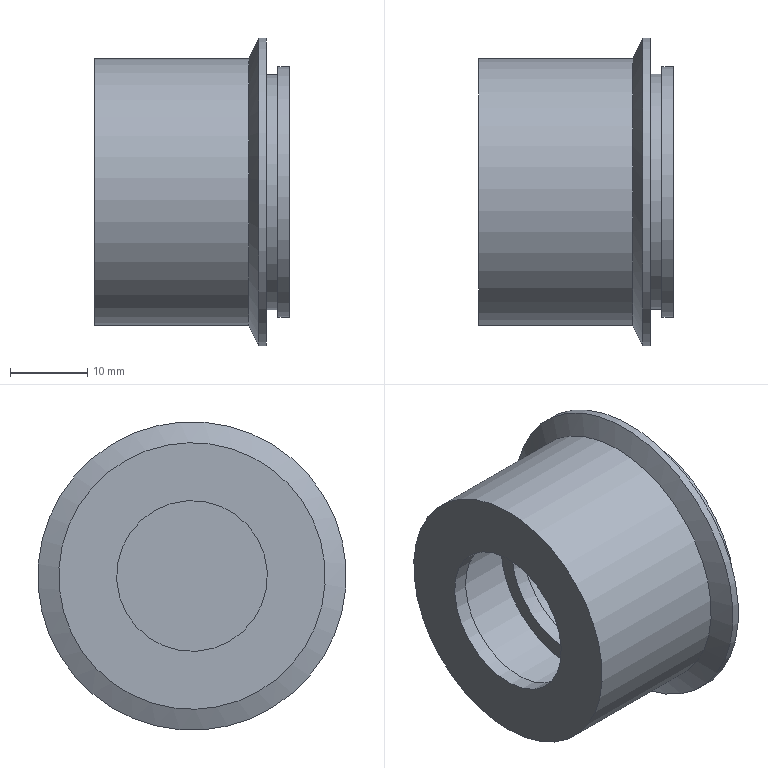Component | NX | VALVE | 1 solid | 19 faces | box 25.27 x 40 x 40 mm | volume 14593 mm3 | plane 9 | cylinder 9 | cone 1 | commonest cylinder face diameters 24.562 x2 19.562 x1 32.562 x1 30.562 x1 40 x1 34.562 x1 20.5 x1 20 x1
STEP:
#1=CARTESIAN_POINT('',(0.,0.,0.));
#2=DIRECTION('',(0.,0.,1.));
#3=DIRECTION('',(1.,0.,0.));
#4=AXIS2_PLACEMENT_3D('',#1,#2,#3);
#5=CARTESIAN_POINT('',(81.232,9.04,3.735));
#6=VERTEX_POINT('',#5);
#7=CARTESIAN_POINT('',(81.232,0.,0.));
#8=DIRECTION('',(-1.,0.,0.));
#9=DIRECTION('',(0.,0.9242,0.3818));
#10=AXIS2_PLACEMENT_3D('',#7,#8,#9);
#11=CIRCLE('',#10,9.781);
#12=CARTESIAN_POINT('',(81.232,-11.35,-4.69));
#13=DIRECTION('',(1.,0.,0.));
#14=DIRECTION('',(0.,-0.9242,-0.3818));
#15=AXIS2_PLACEMENT_3D('',#12,#13,#14);
#16=PLANE('',#15);
#17=CARTESIAN_POINT('',(-22.062,-0.));
#18=CARTESIAN_POINT('',(-22.062,16.941));
#19=CARTESIAN_POINT('',(-7.391,8.471));
#20=CARTESIAN_POINT('',(7.281,-0.));
#21=CARTESIAN_POINT('',(-7.391,-8.471));
#22=CARTESIAN_POINT('',(-22.062,-16.941));
#23=CARTESIAN_POINT('',(-22.062,-0.));
#24=(BOUNDED_CURVE()B_SPLINE_CURVE(2,(#17,#18,#19,#20,#21,#22,#23),.UNSPECIFIED.,.T.,.F.)B_SPLINE_CURVE_WITH_KNOTS((1,2,2,2,2,1),(-2.094,0.,2.094,4.189,6.283,8.378),.UNSPECIFIED.)CURVE()GEOMETRIC_REPRESENTATION_ITEM()RATIONAL_B_SPLINE_CURVE((1.,0.5,1.,0.5,1.,0.5,1.))REPRESENTATION_ITEM(''));
#25=(GEOMETRIC_REPRESENTATION_CONTEXT(2)PARAMETRIC_REPRESENTATION_CONTEXT()REPRESENTATION_CONTEXT('',''));
#26=DEFINITIONAL_REPRESENTATION('',(#24),#25);
#27=PCURVE('',#16,#26);
#28=CARTESIAN_POINT('',(106.5,0.,0.));
#29=DIRECTION('',(-1.,0.,0.));
#30=DIRECTION('',(0.,0.9242,0.3818));
#31=AXIS2_PLACEMENT_3D('',#28,#29,#30);
#32=CYLINDRICAL_SURFACE('',#31,9.781);
#33=CARTESIAN_POINT('',(0.,25.268));
#34=DIRECTION('',(1.,0.));
#35=VECTOR('',#34,1.);
#36=LINE('',#33,#35);
#37=(GEOMETRIC_REPRESENTATION_CONTEXT(2)PARAMETRIC_REPRESENTATION_CONTEXT()REPRESENTATION_CONTEXT('',''));
#38=DEFINITIONAL_REPRESENTATION('',(#36),#37);
#39=PCURVE('',#32,#38);
#40=SURFACE_CURVE('',#11,(#27,#39),.PCURVE_S1.);
#41=EDGE_CURVE('',#6,#6,#40,.T.);
#42=ORIENTED_EDGE('',*,*,#41,.F.);
#43=EDGE_LOOP('',(#42));
#44=FACE_BOUND('',#43,.T.);
#45=CARTESIAN_POINT('',(81.232,15.972,6.599));
#46=VERTEX_POINT('',#45);
#47=CARTESIAN_POINT('',(81.232,0.,0.));
#48=DIRECTION('',(-1.,0.,0.));
#49=DIRECTION('',(0.,0.9242,0.3818));
#50=AXIS2_PLACEMENT_3D('',#47,#48,#49);
#51=CIRCLE('',#50,17.281);
#52=CARTESIAN_POINT('',(-29.562,-0.));
#53=CARTESIAN_POINT('',(-29.562,29.932));
#54=CARTESIAN_POINT('',(-3.641,14.966));
#55=CARTESIAN_POINT('',(22.281,-0.));
#56=CARTESIAN_POINT('',(-3.641,-14.966));
#57=CARTESIAN_POINT('',(-29.562,-29.932));
#58=CARTESIAN_POINT('',(-29.562,-0.));
#59=(BOUNDED_CURVE()B_SPLINE_CURVE(2,(#52,#53,#54,#55,#56,#57,#58),.UNSPECIFIED.,.T.,.F.)B_SPLINE_CURVE_WITH_KNOTS((1,2,2,2,2,1),(-2.094,0.,2.094,4.189,6.283,8.378),.UNSPECIFIED.)CURVE()GEOMETRIC_REPRESENTATION_ITEM()RATIONAL_B_SPLINE_CURVE((1.,0.5,1.,0.5,1.,0.5,1.))REPRESENTATION_ITEM(''));
#60=(GEOMETRIC_REPRESENTATION_CONTEXT(2)PARAMETRIC_REPRESENTATION_CONTEXT()REPRESENTATION_CONTEXT('',''));
#61=DEFINITIONAL_REPRESENTATION('',(#59),#60);
#62=PCURVE('',#16,#61);
#63=CARTESIAN_POINT('',(106.5,0.,0.));
#64=DIRECTION('',(-1.,0.,0.));
#65=DIRECTION('',(0.,0.9242,0.3818));
#66=AXIS2_PLACEMENT_3D('',#63,#64,#65);
#67=CYLINDRICAL_SURFACE('',#66,17.281);
#68=CARTESIAN_POINT('',(0.,25.268));
#69=DIRECTION('',(1.,0.));
#70=VECTOR('',#69,1.);
#71=LINE('',#68,#70);
#72=(GEOMETRIC_REPRESENTATION_CONTEXT(2)PARAMETRIC_REPRESENTATION_CONTEXT()REPRESENTATION_CONTEXT('',''));
#73=DEFINITIONAL_REPRESENTATION('',(#71),#72);
#74=PCURVE('',#67,#73);
#75=SURFACE_CURVE('',#51,(#62,#74),.PCURVE_S1.);
#76=EDGE_CURVE('',#46,#46,#75,.T.);
#77=ORIENTED_EDGE('',*,*,#76,.T.);
#78=EDGE_LOOP('',(#77));
#79=FACE_BOUND('',#78,.T.);
#80=ADVANCED_FACE('',(#44,#79),#16,.F.);
#81=CARTESIAN_POINT('',(83.232,9.04,3.735));
#82=VERTEX_POINT('',#81);
#83=CARTESIAN_POINT('',(83.232,0.,0.));
#84=DIRECTION('',(-1.,0.,0.));
#85=DIRECTION('',(0.,0.9242,0.3818));
#86=AXIS2_PLACEMENT_3D('',#83,#84,#85);
#87=CIRCLE('',#86,9.781);
#88=CARTESIAN_POINT('',(0.,23.268));
#89=DIRECTION('',(1.,0.));
#90=VECTOR('',#89,1.);
#91=LINE('',#88,#90);
#92=(GEOMETRIC_REPRESENTATION_CONTEXT(2)PARAMETRIC_REPRESENTATION_CONTEXT()REPRESENTATION_CONTEXT('',''));
#93=DEFINITIONAL_REPRESENTATION('',(#91),#92);
#94=PCURVE('',#32,#93);
#95=CARTESIAN_POINT('',(83.232,-9.04,-3.735));
#96=DIRECTION('',(-1.,0.,0.));
#97=DIRECTION('',(0.,0.9242,0.3818));
#98=AXIS2_PLACEMENT_3D('',#95,#96,#97);
#99=PLANE('',#98);
#100=CARTESIAN_POINT('',(9.781,0.));
#101=DIRECTION('',(1.,0.));
#102=AXIS2_PLACEMENT_2D('',#100,#101);
#103=CIRCLE('',#102,9.781);
#104=(GEOMETRIC_REPRESENTATION_CONTEXT(2)PARAMETRIC_REPRESENTATION_CONTEXT()REPRESENTATION_CONTEXT('',''));
#105=DEFINITIONAL_REPRESENTATION('',(#103),#104);
#106=PCURVE('',#99,#105);
#107=SURFACE_CURVE('',#87,(#94,#106),.PCURVE_S1.);
#108=EDGE_CURVE('',#82,#82,#107,.T.);
#109=ORIENTED_EDGE('',*,*,#108,.T.);
#110=CARTESIAN_POINT('',(83.232,9.04,3.735));
#111=CARTESIAN_POINT('',(81.232,9.04,3.735));
#112=B_SPLINE_CURVE_WITH_KNOTS('',1,(#110,#111),.UNSPECIFIED.,.F.,.F.,(2,2),(23.268,25.268),.PIECEWISE_BEZIER_KNOTS.);
#113=CARTESIAN_POINT('',(6.283,0.));
#114=DIRECTION('',(0.,1.));
#115=VECTOR('',#114,1.);
#116=LINE('',#113,#115);
#117=(GEOMETRIC_REPRESENTATION_CONTEXT(2)PARAMETRIC_REPRESENTATION_CONTEXT()REPRESENTATION_CONTEXT('',''));
#118=DEFINITIONAL_REPRESENTATION('',(#116),#117);
#119=PCURVE('',#32,#118);
#120=CARTESIAN_POINT('',(0.,0.));
#121=DIRECTION('',(0.,1.));
#122=VECTOR('',#121,1.);
#123=LINE('',#120,#122);
#124=(GEOMETRIC_REPRESENTATION_CONTEXT(2)PARAMETRIC_REPRESENTATION_CONTEXT()REPRESENTATION_CONTEXT('',''));
#125=DEFINITIONAL_REPRESENTATION('',(#123),#124);
#126=PCURVE('',#32,#125);
#127=SEAM_CURVE('',#112,(#119,#126),.PCURVE_S1.);
#128=EDGE_CURVE('',#82,#6,#127,.T.);
#129=ORIENTED_EDGE('',*,*,#128,.T.);
#130=ORIENTED_EDGE('',*,*,#41,.F.);
#131=ORIENTED_EDGE('',*,*,#128,.F.);
#132=EDGE_LOOP('',(#109,#129,#130,#131));
#133=FACE_BOUND('',#132,.F.);
#134=ADVANCED_FACE('',(#133),#32,.F.);
#135=CARTESIAN_POINT('',(83.232,11.35,4.69));
#136=VERTEX_POINT('',#135);
#137=CARTESIAN_POINT('',(83.232,0.,0.));
#138=DIRECTION('',(-1.,0.,0.));
#139=DIRECTION('',(0.,0.9242,0.3818));
#140=AXIS2_PLACEMENT_3D('',#137,#138,#139);
#141=CIRCLE('',#140,12.281);
#142=CARTESIAN_POINT('',(9.781,0.));
#143=DIRECTION('',(1.,-0.));
#144=AXIS2_PLACEMENT_2D('',#142,#143);
#145=CIRCLE('',#144,12.281);
#146=(GEOMETRIC_REPRESENTATION_CONTEXT(2)PARAMETRIC_REPRESENTATION_CONTEXT()REPRESENTATION_CONTEXT('',''));
#147=DEFINITIONAL_REPRESENTATION('',(#145),#146);
#148=PCURVE('',#99,#147);
#149=CARTESIAN_POINT('',(106.5,0.,0.));
#150=DIRECTION('',(-1.,0.,0.));
#151=DIRECTION('',(0.,0.9242,0.3818));
#152=AXIS2_PLACEMENT_3D('',#149,#150,#151);
#153=CYLINDRICAL_SURFACE('',#152,12.281);
#154=CARTESIAN_POINT('',(0.,23.268));
#155=DIRECTION('',(1.,0.));
#156=VECTOR('',#155,1.);
#157=LINE('',#154,#156);
#158=(GEOMETRIC_REPRESENTATION_CONTEXT(2)PARAMETRIC_REPRESENTATION_CONTEXT()REPRESENTATION_CONTEXT('',''));
#159=DEFINITIONAL_REPRESENTATION('',(#157),#158);
#160=PCURVE('',#153,#159);
#161=SURFACE_CURVE('',#141,(#148,#160),.PCURVE_S1.);
#162=EDGE_CURVE('',#136,#136,#161,.T.);
#163=ORIENTED_EDGE('',*,*,#162,.F.);
#164=EDGE_LOOP('',(#163));
#165=FACE_BOUND('',#164,.T.);
#166=ORIENTED_EDGE('',*,*,#108,.T.);
#167=EDGE_LOOP('',(#166));
#168=FACE_BOUND('',#167,.T.);
#169=ADVANCED_FACE('',(#165,#168),#99,.F.);
#170=CARTESIAN_POINT('',(92.232,11.35,4.69));
#171=VERTEX_POINT('',#170);
#172=CARTESIAN_POINT('',(92.232,0.,0.));
#173=DIRECTION('',(-1.,0.,0.));
#174=DIRECTION('',(0.,0.9242,0.3818));
#175=AXIS2_PLACEMENT_3D('',#172,#173,#174);
#176=CIRCLE('',#175,12.281);
#177=CARTESIAN_POINT('',(0.,14.268));
#178=DIRECTION('',(1.,0.));
#179=VECTOR('',#178,1.);
#180=LINE('',#177,#179);
#181=(GEOMETRIC_REPRESENTATION_CONTEXT(2)PARAMETRIC_REPRESENTATION_CONTEXT()REPRESENTATION_CONTEXT('',''));
#182=DEFINITIONAL_REPRESENTATION('',(#180),#181);
#183=PCURVE('',#153,#182);
#184=CARTESIAN_POINT('',(92.232,-11.35,-4.69));
#185=DIRECTION('',(1.,0.,0.));
#186=DIRECTION('',(0.,-0.9242,-0.3818));
#187=AXIS2_PLACEMENT_3D('',#184,#185,#186);
#188=PLANE('',#187);
#189=CARTESIAN_POINT('',(-24.562,-0.));
#190=CARTESIAN_POINT('',(-24.562,21.271));
#191=CARTESIAN_POINT('',(-6.141,10.636));
#192=CARTESIAN_POINT('',(12.281,0.));
#193=CARTESIAN_POINT('',(-6.141,-10.636));
#194=CARTESIAN_POINT('',(-24.562,-21.271));
#195=CARTESIAN_POINT('',(-24.562,-0.));
#196=(BOUNDED_CURVE()B_SPLINE_CURVE(2,(#189,#190,#191,#192,#193,#194,#195),.UNSPECIFIED.,.T.,.F.)B_SPLINE_CURVE_WITH_KNOTS((1,2,2,2,2,1),(-2.094,0.,2.094,4.189,6.283,8.378),.UNSPECIFIED.)CURVE()GEOMETRIC_REPRESENTATION_ITEM()RATIONAL_B_SPLINE_CURVE((1.,0.5,1.,0.5,1.,0.5,1.))REPRESENTATION_ITEM(''));
#197=(GEOMETRIC_REPRESENTATION_CONTEXT(2)PARAMETRIC_REPRESENTATION_CONTEXT()REPRESENTATION_CONTEXT('',''));
#198=DEFINITIONAL_REPRESENTATION('',(#196),#197);
#199=PCURVE('',#188,#198);
#200=SURFACE_CURVE('',#176,(#183,#199),.PCURVE_S1.);
#201=EDGE_CURVE('',#171,#171,#200,.T.);
#202=ORIENTED_EDGE('',*,*,#201,.T.);
#203=CARTESIAN_POINT('',(92.232,11.35,4.69));
#204=CARTESIAN_POINT('',(83.232,11.35,4.69));
#205=B_SPLINE_CURVE_WITH_KNOTS('',1,(#203,#204),.UNSPECIFIED.,.F.,.F.,(2,2),(14.268,23.268),.PIECEWISE_BEZIER_KNOTS.);
#206=CARTESIAN_POINT('',(6.283,0.));
#207=DIRECTION('',(0.,1.));
#208=VECTOR('',#207,1.);
#209=LINE('',#206,#208);
#210=(GEOMETRIC_REPRESENTATION_CONTEXT(2)PARAMETRIC_REPRESENTATION_CONTEXT()REPRESENTATION_CONTEXT('',''));
#211=DEFINITIONAL_REPRESENTATION('',(#209),#210);
#212=PCURVE('',#153,#211);
#213=CARTESIAN_POINT('',(0.,0.));
#214=DIRECTION('',(0.,1.));
#215=VECTOR('',#214,1.);
#216=LINE('',#213,#215);
#217=(GEOMETRIC_REPRESENTATION_CONTEXT(2)PARAMETRIC_REPRESENTATION_CONTEXT()REPRESENTATION_CONTEXT('',''));
#218=DEFINITIONAL_REPRESENTATION('',(#216),#217);
#219=PCURVE('',#153,#218);
#220=SEAM_CURVE('',#205,(#212,#219),.PCURVE_S1.);
#221=EDGE_CURVE('',#171,#136,#220,.T.);
#222=ORIENTED_EDGE('',*,*,#221,.T.);
#223=ORIENTED_EDGE('',*,*,#162,.F.);
#224=ORIENTED_EDGE('',*,*,#221,.F.);
#225=EDGE_LOOP('',(#202,#222,#223,#224));
#226=FACE_BOUND('',#225,.F.);
#227=ADVANCED_FACE('',(#226),#153,.F.);
#228=CARTESIAN_POINT('',(92.232,-9.473,-3.914));
#229=VERTEX_POINT('',#228);
#230=CARTESIAN_POINT('',(92.232,9.473,3.914));
#231=VERTEX_POINT('',#230);
#232=CARTESIAN_POINT('',(92.232,0.,0.));
#233=DIRECTION('',(1.,0.,0.));
#234=DIRECTION('',(0.,-0.9242,-0.3818));
#235=AXIS2_PLACEMENT_3D('',#232,#233,#234);
#236=CIRCLE('',#235,10.25);
#237=CARTESIAN_POINT('',(-12.281,-0.));
#238=DIRECTION('',(1.,0.));
#239=AXIS2_PLACEMENT_2D('',#237,#238);
#240=CIRCLE('',#239,10.25);
#241=(GEOMETRIC_REPRESENTATION_CONTEXT(2)PARAMETRIC_REPRESENTATION_CONTEXT()REPRESENTATION_CONTEXT('',''));
#242=DEFINITIONAL_REPRESENTATION('',(#240),#241);
#243=PCURVE('',#188,#242);
#244=CARTESIAN_POINT('',(92.,0.,0.));
#245=DIRECTION('',(1.,0.,0.));
#246=DIRECTION('',(0.,0.3818,-0.9242));
#247=AXIS2_PLACEMENT_3D('',#244,#245,#246);
#248=CYLINDRICAL_SURFACE('',#247,10.25);
#249=CARTESIAN_POINT('',(4.712,0.2321));
#250=DIRECTION('',(1.,0.));
#251=VECTOR('',#250,1.);
#252=LINE('',#249,#251);
#253=(GEOMETRIC_REPRESENTATION_CONTEXT(2)PARAMETRIC_REPRESENTATION_CONTEXT()REPRESENTATION_CONTEXT('',''));
#254=DEFINITIONAL_REPRESENTATION('',(#252),#253);
#255=PCURVE('',#248,#254);
#256=SURFACE_CURVE('',#236,(#243,#255),.PCURVE_S1.);
#257=EDGE_CURVE('',#229,#231,#256,.T.);
#258=ORIENTED_EDGE('',*,*,#257,.T.);
#259=CARTESIAN_POINT('',(92.232,0.,0.));
#260=DIRECTION('',(1.,0.,0.));
#261=DIRECTION('',(0.,-0.9242,-0.3818));
#262=AXIS2_PLACEMENT_3D('',#259,#260,#261);
#263=CIRCLE('',#262,10.25);
#264=CARTESIAN_POINT('',(-12.281,-0.));
#265=DIRECTION('',(1.,0.));
#266=AXIS2_PLACEMENT_2D('',#264,#265);
#267=CIRCLE('',#266,10.25);
#268=(GEOMETRIC_REPRESENTATION_CONTEXT(2)PARAMETRIC_REPRESENTATION_CONTEXT()REPRESENTATION_CONTEXT('',''));
#269=DEFINITIONAL_REPRESENTATION('',(#267),#268);
#270=PCURVE('',#188,#269);
#271=CARTESIAN_POINT('',(-1.571,0.2321));
#272=DIRECTION('',(1.,0.));
#273=VECTOR('',#272,1.);
#274=LINE('',#271,#273);
#275=(GEOMETRIC_REPRESENTATION_CONTEXT(2)PARAMETRIC_REPRESENTATION_CONTEXT()REPRESENTATION_CONTEXT('',''));
#276=DEFINITIONAL_REPRESENTATION('',(#274),#275);
#277=PCURVE('',#248,#276);
#278=SURFACE_CURVE('',#263,(#270,#277),.PCURVE_S1.);
#279=EDGE_CURVE('',#231,#229,#278,.T.);
#280=ORIENTED_EDGE('',*,*,#279,.T.);
#281=EDGE_LOOP('',(#258,#280));
#282=FACE_BOUND('',#281,.T.);
#283=ORIENTED_EDGE('',*,*,#201,.T.);
#284=EDGE_LOOP('',(#283));
#285=FACE_BOUND('',#284,.T.);
#286=ADVANCED_FACE('',(#282,#285),#188,.F.);
#287=CARTESIAN_POINT('',(106.5,15.047,6.217));
#288=VERTEX_POINT('',#287);
#289=CARTESIAN_POINT('',(106.5,0.,0.));
#290=DIRECTION('',(-1.,0.,0.));
#291=DIRECTION('',(0.,0.9242,0.3818));
#292=AXIS2_PLACEMENT_3D('',#289,#290,#291);
#293=CIRCLE('',#292,16.281);
#294=CARTESIAN_POINT('',(106.5,0.,0.));
#295=DIRECTION('',(-1.,0.,0.));
#296=DIRECTION('',(0.,0.9242,0.3818));
#297=AXIS2_PLACEMENT_3D('',#294,#295,#296);
#298=PLANE('',#297);
#299=CARTESIAN_POINT('',(0.,0.));
#300=DIRECTION('',(1.,0.));
#301=AXIS2_PLACEMENT_2D('',#299,#300);
#302=CIRCLE('',#301,16.281);
#303=(GEOMETRIC_REPRESENTATION_CONTEXT(2)PARAMETRIC_REPRESENTATION_CONTEXT()REPRESENTATION_CONTEXT('',''));
#304=DEFINITIONAL_REPRESENTATION('',(#302),#303);
#305=PCURVE('',#298,#304);
#306=CARTESIAN_POINT('',(106.5,0.,0.));
#307=DIRECTION('',(-1.,0.,0.));
#308=DIRECTION('',(0.,0.9242,0.3818));
#309=AXIS2_PLACEMENT_3D('',#306,#307,#308);
#310=CYLINDRICAL_SURFACE('',#309,16.281);
#311=CARTESIAN_POINT('',(0.,0.));
#312=DIRECTION('',(1.,0.));
#313=VECTOR('',#312,1.);
#314=LINE('',#311,#313);
#315=(GEOMETRIC_REPRESENTATION_CONTEXT(2)PARAMETRIC_REPRESENTATION_CONTEXT()REPRESENTATION_CONTEXT('',''));
#316=DEFINITIONAL_REPRESENTATION('',(#314),#315);
#317=PCURVE('',#310,#316);
#318=SURFACE_CURVE('',#293,(#305,#317),.PCURVE_S1.);
#319=EDGE_CURVE('',#288,#288,#318,.T.);
#320=ORIENTED_EDGE('',*,*,#319,.F.);
#321=EDGE_LOOP('',(#320));
#322=FACE_BOUND('',#321,.T.);
#323=ADVANCED_FACE('',(#322),#298,.F.);
#324=CARTESIAN_POINT('',(105.,15.047,6.217));
#325=VERTEX_POINT('',#324);
#326=CARTESIAN_POINT('',(105.,0.,0.));
#327=DIRECTION('',(-1.,0.,0.));
#328=DIRECTION('',(0.,0.9242,0.3818));
#329=AXIS2_PLACEMENT_3D('',#326,#327,#328);
#330=CIRCLE('',#329,16.281);
#331=CARTESIAN_POINT('',(0.,1.5));
#332=DIRECTION('',(1.,0.));
#333=VECTOR('',#332,1.);
#334=LINE('',#331,#333);
#335=(GEOMETRIC_REPRESENTATION_CONTEXT(2)PARAMETRIC_REPRESENTATION_CONTEXT()REPRESENTATION_CONTEXT('',''));
#336=DEFINITIONAL_REPRESENTATION('',(#334),#335);
#337=PCURVE('',#310,#336);
#338=CARTESIAN_POINT('',(105.,-15.047,-6.217));
#339=DIRECTION('',(1.,0.,0.));
#340=DIRECTION('',(0.,-0.9242,-0.3818));
#341=AXIS2_PLACEMENT_3D('',#338,#339,#340);
#342=PLANE('',#341);
#343=CARTESIAN_POINT('',(-32.562,-0.));
#344=CARTESIAN_POINT('',(-32.562,28.2));
#345=CARTESIAN_POINT('',(-8.141,14.1));
#346=CARTESIAN_POINT('',(16.281,-0.));
#347=CARTESIAN_POINT('',(-8.141,-14.1));
#348=CARTESIAN_POINT('',(-32.562,-28.2));
#349=CARTESIAN_POINT('',(-32.562,-0.));
#350=(BOUNDED_CURVE()B_SPLINE_CURVE(2,(#343,#344,#345,#346,#347,#348,#349),.UNSPECIFIED.,.T.,.F.)B_SPLINE_CURVE_WITH_KNOTS((1,2,2,2,2,1),(-2.094,0.,2.094,4.189,6.283,8.378),.UNSPECIFIED.)CURVE()GEOMETRIC_REPRESENTATION_ITEM()RATIONAL_B_SPLINE_CURVE((1.,0.5,1.,0.5,1.,0.5,1.))REPRESENTATION_ITEM(''));
#351=(GEOMETRIC_REPRESENTATION_CONTEXT(2)PARAMETRIC_REPRESENTATION_CONTEXT()REPRESENTATION_CONTEXT('',''));
#352=DEFINITIONAL_REPRESENTATION('',(#350),#351);
#353=PCURVE('',#342,#352);
#354=SURFACE_CURVE('',#330,(#337,#353),.PCURVE_S1.);
#355=EDGE_CURVE('',#325,#325,#354,.T.);
#356=ORIENTED_EDGE('',*,*,#355,.F.);
#357=CARTESIAN_POINT('',(106.5,15.047,6.217));
#358=CARTESIAN_POINT('',(105.,15.047,6.217));
#359=B_SPLINE_CURVE_WITH_KNOTS('',1,(#357,#358),.UNSPECIFIED.,.F.,.F.,(2,2),(0.,1.5),.PIECEWISE_BEZIER_KNOTS.);
#360=CARTESIAN_POINT('',(0.,0.));
#361=DIRECTION('',(0.,1.));
#362=VECTOR('',#361,1.);
#363=LINE('',#360,#362);
#364=(GEOMETRIC_REPRESENTATION_CONTEXT(2)PARAMETRIC_REPRESENTATION_CONTEXT()REPRESENTATION_CONTEXT('',''));
#365=DEFINITIONAL_REPRESENTATION('',(#363),#364);
#366=PCURVE('',#310,#365);
#367=CARTESIAN_POINT('',(6.283,0.));
#368=DIRECTION('',(0.,1.));
#369=VECTOR('',#368,1.);
#370=LINE('',#367,#369);
#371=(GEOMETRIC_REPRESENTATION_CONTEXT(2)PARAMETRIC_REPRESENTATION_CONTEXT()REPRESENTATION_CONTEXT('',''));
#372=DEFINITIONAL_REPRESENTATION('',(#370),#371);
#373=PCURVE('',#310,#372);
#374=SEAM_CURVE('',#359,(#366,#373),.PCURVE_S1.);
#375=EDGE_CURVE('',#288,#325,#374,.T.);
#376=ORIENTED_EDGE('',*,*,#375,.F.);
#377=ORIENTED_EDGE('',*,*,#319,.T.);
#378=ORIENTED_EDGE('',*,*,#375,.T.);
#379=EDGE_LOOP('',(#356,#376,#377,#378));
#380=FACE_BOUND('',#379,.T.);
#381=ADVANCED_FACE('',(#380),#310,.T.);
#382=CARTESIAN_POINT('',(105.,14.123,5.835));
#383=VERTEX_POINT('',#382);
#384=CARTESIAN_POINT('',(105.,0.,0.));
#385=DIRECTION('',(-1.,0.,0.));
#386=DIRECTION('',(0.,0.9242,0.3818));
#387=AXIS2_PLACEMENT_3D('',#384,#385,#386);
#388=CIRCLE('',#387,15.281);
#389=CARTESIAN_POINT('',(-31.562,-0.));
#390=CARTESIAN_POINT('',(-31.562,26.468));
#391=CARTESIAN_POINT('',(-8.641,13.234));
#392=CARTESIAN_POINT('',(14.281,-0.));
#393=CARTESIAN_POINT('',(-8.641,-13.234));
#394=CARTESIAN_POINT('',(-31.562,-26.468));
#395=CARTESIAN_POINT('',(-31.562,-0.));
#396=(BOUNDED_CURVE()B_SPLINE_CURVE(2,(#389,#390,#391,#392,#393,#394,#395),.UNSPECIFIED.,.T.,.F.)B_SPLINE_CURVE_WITH_KNOTS((1,2,2,2,2,1),(-2.094,0.,2.094,4.189,6.283,8.378),.UNSPECIFIED.)CURVE()GEOMETRIC_REPRESENTATION_ITEM()RATIONAL_B_SPLINE_CURVE((1.,0.5,1.,0.5,1.,0.5,1.))REPRESENTATION_ITEM(''));
#397=(GEOMETRIC_REPRESENTATION_CONTEXT(2)PARAMETRIC_REPRESENTATION_CONTEXT()REPRESENTATION_CONTEXT('',''));
#398=DEFINITIONAL_REPRESENTATION('',(#396),#397);
#399=PCURVE('',#342,#398);
#400=CARTESIAN_POINT('',(106.5,0.,0.));
#401=DIRECTION('',(-1.,0.,0.));
#402=DIRECTION('',(0.,0.9242,0.3818));
#403=AXIS2_PLACEMENT_3D('',#400,#401,#402);
#404=CYLINDRICAL_SURFACE('',#403,15.281);
#405=CARTESIAN_POINT('',(0.,1.5));
#406=DIRECTION('',(1.,0.));
#407=VECTOR('',#406,1.);
#408=LINE('',#405,#407);
#409=(GEOMETRIC_REPRESENTATION_CONTEXT(2)PARAMETRIC_REPRESENTATION_CONTEXT()REPRESENTATION_CONTEXT('',''));
#410=DEFINITIONAL_REPRESENTATION('',(#408),#409);
#411=PCURVE('',#404,#410);
#412=SURFACE_CURVE('',#388,(#399,#411),.PCURVE_S1.);
#413=EDGE_CURVE('',#383,#383,#412,.T.);
#414=ORIENTED_EDGE('',*,*,#413,.F.);
#415=EDGE_LOOP('',(#414));
#416=FACE_BOUND('',#415,.T.);
#417=ORIENTED_EDGE('',*,*,#355,.T.);
#418=EDGE_LOOP('',(#417));
#419=FACE_BOUND('',#418,.T.);
#420=ADVANCED_FACE('',(#416,#419),#342,.F.);
#421=CARTESIAN_POINT('',(103.5,14.123,5.835));
#422=VERTEX_POINT('',#421);
#423=CARTESIAN_POINT('',(103.5,0.,0.));
#424=DIRECTION('',(-1.,0.,0.));
#425=DIRECTION('',(0.,0.9242,0.3818));
#426=AXIS2_PLACEMENT_3D('',#423,#424,#425);
#427=CIRCLE('',#426,15.281);
#428=CARTESIAN_POINT('',(0.,3.));
#429=DIRECTION('',(1.,0.));
#430=VECTOR('',#429,1.);
#431=LINE('',#428,#430);
#432=(GEOMETRIC_REPRESENTATION_CONTEXT(2)PARAMETRIC_REPRESENTATION_CONTEXT()REPRESENTATION_CONTEXT('',''));
#433=DEFINITIONAL_REPRESENTATION('',(#431),#432);
#434=PCURVE('',#404,#433);
#435=CARTESIAN_POINT('',(103.5,-15.047,-6.217));
#436=DIRECTION('',(-1.,0.,0.));
#437=DIRECTION('',(0.,0.9242,0.3818));
#438=AXIS2_PLACEMENT_3D('',#435,#436,#437);
#439=PLANE('',#438);
#440=CARTESIAN_POINT('',(16.281,-0.));
#441=DIRECTION('',(1.,0.));
#442=AXIS2_PLACEMENT_2D('',#440,#441);
#443=CIRCLE('',#442,15.281);
#444=(GEOMETRIC_REPRESENTATION_CONTEXT(2)PARAMETRIC_REPRESENTATION_CONTEXT()REPRESENTATION_CONTEXT('',''));
#445=DEFINITIONAL_REPRESENTATION('',(#443),#444);
#446=PCURVE('',#439,#445);
#447=SURFACE_CURVE('',#427,(#434,#446),.PCURVE_S1.);
#448=EDGE_CURVE('',#422,#422,#447,.T.);
#449=ORIENTED_EDGE('',*,*,#448,.F.);
#450=CARTESIAN_POINT('',(105.,14.123,5.835));
#451=CARTESIAN_POINT('',(103.5,14.123,5.835));
#452=B_SPLINE_CURVE_WITH_KNOTS('',1,(#450,#451),.UNSPECIFIED.,.F.,.F.,(2,2),(1.5,3.),.PIECEWISE_BEZIER_KNOTS.);
#453=CARTESIAN_POINT('',(0.,0.));
#454=DIRECTION('',(0.,1.));
#455=VECTOR('',#454,1.);
#456=LINE('',#453,#455);
#457=(GEOMETRIC_REPRESENTATION_CONTEXT(2)PARAMETRIC_REPRESENTATION_CONTEXT()REPRESENTATION_CONTEXT('',''));
#458=DEFINITIONAL_REPRESENTATION('',(#456),#457);
#459=PCURVE('',#404,#458);
#460=CARTESIAN_POINT('',(6.283,0.));
#461=DIRECTION('',(0.,1.));
#462=VECTOR('',#461,1.);
#463=LINE('',#460,#462);
#464=(GEOMETRIC_REPRESENTATION_CONTEXT(2)PARAMETRIC_REPRESENTATION_CONTEXT()REPRESENTATION_CONTEXT('',''));
#465=DEFINITIONAL_REPRESENTATION('',(#463),#464);
#466=PCURVE('',#404,#465);
#467=SEAM_CURVE('',#452,(#459,#466),.PCURVE_S1.);
#468=EDGE_CURVE('',#383,#422,#467,.T.);
#469=ORIENTED_EDGE('',*,*,#468,.F.);
#470=ORIENTED_EDGE('',*,*,#413,.T.);
#471=ORIENTED_EDGE('',*,*,#468,.T.);
#472=EDGE_LOOP('',(#449,#469,#470,#471));
#473=FACE_BOUND('',#472,.T.);
#474=ADVANCED_FACE('',(#473),#404,.T.);
#475=CARTESIAN_POINT('',(103.5,18.484,7.637));
#476=VERTEX_POINT('',#475);
#477=CARTESIAN_POINT('',(103.5,0.,0.));
#478=DIRECTION('',(-1.,0.,0.));
#479=DIRECTION('',(0.,0.9242,0.3818));
#480=AXIS2_PLACEMENT_3D('',#477,#478,#479);
#481=CIRCLE('',#480,20.);
#482=CARTESIAN_POINT('',(16.281,-0.));
#483=DIRECTION('',(1.,0.));
#484=AXIS2_PLACEMENT_2D('',#482,#483);
#485=CIRCLE('',#484,20.);
#486=(GEOMETRIC_REPRESENTATION_CONTEXT(2)PARAMETRIC_REPRESENTATION_CONTEXT()REPRESENTATION_CONTEXT('',''));
#487=DEFINITIONAL_REPRESENTATION('',(#485),#486);
#488=PCURVE('',#439,#487);
#489=CARTESIAN_POINT('',(106.5,0.,0.));
#490=DIRECTION('',(-1.,0.,0.));
#491=DIRECTION('',(0.,0.9242,0.3818));
#492=AXIS2_PLACEMENT_3D('',#489,#490,#491);
#493=CYLINDRICAL_SURFACE('',#492,20.);
#494=CARTESIAN_POINT('',(0.,3.));
#495=DIRECTION('',(1.,0.));
#496=VECTOR('',#495,1.);
#497=LINE('',#494,#496);
#498=(GEOMETRIC_REPRESENTATION_CONTEXT(2)PARAMETRIC_REPRESENTATION_CONTEXT()REPRESENTATION_CONTEXT('',''));
#499=DEFINITIONAL_REPRESENTATION('',(#497),#498);
#500=PCURVE('',#493,#499);
#501=SURFACE_CURVE('',#481,(#488,#500),.PCURVE_S1.);
#502=EDGE_CURVE('',#476,#476,#501,.T.);
#503=ORIENTED_EDGE('',*,*,#502,.F.);
#504=EDGE_LOOP('',(#503));
#505=FACE_BOUND('',#504,.T.);
#506=ORIENTED_EDGE('',*,*,#448,.T.);
#507=EDGE_LOOP('',(#506));
#508=FACE_BOUND('',#507,.T.);
#509=ADVANCED_FACE('',(#505,#508),#439,.F.);
#510=CARTESIAN_POINT('',(102.5,18.484,7.637));
#511=VERTEX_POINT('',#510);
#512=CARTESIAN_POINT('',(102.5,0.,0.));
#513=DIRECTION('',(-1.,0.,0.));
#514=DIRECTION('',(0.,0.9242,0.3818));
#515=AXIS2_PLACEMENT_3D('',#512,#513,#514);
#516=CIRCLE('',#515,20.);
#517=CARTESIAN_POINT('',(0.,4.));
#518=DIRECTION('',(1.,0.));
#519=VECTOR('',#518,1.);
#520=LINE('',#517,#519);
#521=(GEOMETRIC_REPRESENTATION_CONTEXT(2)PARAMETRIC_REPRESENTATION_CONTEXT()REPRESENTATION_CONTEXT('',''));
#522=DEFINITIONAL_REPRESENTATION('',(#520),#521);
#523=PCURVE('',#493,#522);
#524=CARTESIAN_POINT('',(102.5,0.,0.));
#525=DIRECTION('',(1.,0.,0.));
#526=DIRECTION('',(0.,-0.9242,-0.3818));
#527=AXIS2_PLACEMENT_3D('',#524,#525,#526);
#528=CONICAL_SURFACE('',#527,20.,1.134);
#529=CARTESIAN_POINT('',(9.425,0.));
#530=DIRECTION('',(-1.,-0.));
#531=VECTOR('',#530,1.);
#532=LINE('',#529,#531);
#533=(GEOMETRIC_REPRESENTATION_CONTEXT(2)PARAMETRIC_REPRESENTATION_CONTEXT()REPRESENTATION_CONTEXT('',''));
#534=DEFINITIONAL_REPRESENTATION('',(#532),#533);
#535=PCURVE('',#528,#534);
#536=SURFACE_CURVE('',#516,(#523,#535),.PCURVE_S1.);
#537=EDGE_CURVE('',#511,#511,#536,.T.);
#538=ORIENTED_EDGE('',*,*,#537,.F.);
#539=CARTESIAN_POINT('',(103.5,18.484,7.637));
#540=CARTESIAN_POINT('',(102.5,18.484,7.637));
#541=B_SPLINE_CURVE_WITH_KNOTS('',1,(#539,#540),.UNSPECIFIED.,.F.,.F.,(2,2),(3.,4.),.PIECEWISE_BEZIER_KNOTS.);
#542=CARTESIAN_POINT('',(0.,0.));
#543=DIRECTION('',(0.,1.));
#544=VECTOR('',#543,1.);
#545=LINE('',#542,#544);
#546=(GEOMETRIC_REPRESENTATION_CONTEXT(2)PARAMETRIC_REPRESENTATION_CONTEXT()REPRESENTATION_CONTEXT('',''));
#547=DEFINITIONAL_REPRESENTATION('',(#545),#546);
#548=PCURVE('',#493,#547);
#549=CARTESIAN_POINT('',(6.283,0.));
#550=DIRECTION('',(0.,1.));
#551=VECTOR('',#550,1.);
#552=LINE('',#549,#551);
#553=(GEOMETRIC_REPRESENTATION_CONTEXT(2)PARAMETRIC_REPRESENTATION_CONTEXT()REPRESENTATION_CONTEXT('',''));
#554=DEFINITIONAL_REPRESENTATION('',(#552),#553);
#555=PCURVE('',#493,#554);
#556=SEAM_CURVE('',#541,(#548,#555),.PCURVE_S1.);
#557=EDGE_CURVE('',#476,#511,#556,.T.);
#558=ORIENTED_EDGE('',*,*,#557,.F.);
#559=ORIENTED_EDGE('',*,*,#502,.T.);
#560=ORIENTED_EDGE('',*,*,#557,.T.);
#561=EDGE_LOOP('',(#538,#558,#559,#560));
#562=FACE_BOUND('',#561,.T.);
#563=ADVANCED_FACE('',(#562),#493,.T.);
#564=CARTESIAN_POINT('',(101.232,15.972,6.599));
#565=VERTEX_POINT('',#564);
#566=CARTESIAN_POINT('',(101.232,0.,0.));
#567=DIRECTION('',(-1.,0.,0.));
#568=DIRECTION('',(0.,0.9242,0.3818));
#569=AXIS2_PLACEMENT_3D('',#566,#567,#568);
#570=CIRCLE('',#569,17.281);
#571=CARTESIAN_POINT('',(9.425,-1.268));
#572=DIRECTION('',(-1.,0.));
#573=VECTOR('',#572,1.);
#574=LINE('',#571,#573);
#575=(GEOMETRIC_REPRESENTATION_CONTEXT(2)PARAMETRIC_REPRESENTATION_CONTEXT()REPRESENTATION_CONTEXT('',''));
#576=DEFINITIONAL_REPRESENTATION('',(#574),#575);
#577=PCURVE('',#528,#576);
#578=CARTESIAN_POINT('',(0.,5.268));
#579=DIRECTION('',(1.,0.));
#580=VECTOR('',#579,1.);
#581=LINE('',#578,#580);
#582=(GEOMETRIC_REPRESENTATION_CONTEXT(2)PARAMETRIC_REPRESENTATION_CONTEXT()REPRESENTATION_CONTEXT('',''));
#583=DEFINITIONAL_REPRESENTATION('',(#581),#582);
#584=PCURVE('',#67,#583);
#585=SURFACE_CURVE('',#570,(#577,#584),.PCURVE_S1.);
#586=EDGE_CURVE('',#565,#565,#585,.T.);
#587=ORIENTED_EDGE('',*,*,#586,.F.);
#588=CARTESIAN_POINT('',(101.232,15.972,6.599));
#589=CARTESIAN_POINT('',(102.5,18.484,7.637));
#590=B_SPLINE_CURVE_WITH_KNOTS('',1,(#588,#589),.UNSPECIFIED.,.F.,.F.,(2,2),(-3.,-0.),.PIECEWISE_BEZIER_KNOTS.);
#591=CARTESIAN_POINT('',(9.425,0.));
#592=DIRECTION('',(0.,1.));
#593=VECTOR('',#592,1.);
#594=LINE('',#591,#593);
#595=(GEOMETRIC_REPRESENTATION_CONTEXT(2)PARAMETRIC_REPRESENTATION_CONTEXT()REPRESENTATION_CONTEXT('',''));
#596=DEFINITIONAL_REPRESENTATION('',(#594),#595);
#597=PCURVE('',#528,#596);
#598=CARTESIAN_POINT('',(3.142,0.));
#599=DIRECTION('',(0.,1.));
#600=VECTOR('',#599,1.);
#601=LINE('',#598,#600);
#602=(GEOMETRIC_REPRESENTATION_CONTEXT(2)PARAMETRIC_REPRESENTATION_CONTEXT()REPRESENTATION_CONTEXT('',''));
#603=DEFINITIONAL_REPRESENTATION('',(#601),#602);
#604=PCURVE('',#528,#603);
#605=SEAM_CURVE('',#590,(#597,#604),.PCURVE_S1.);
#606=EDGE_CURVE('',#565,#511,#605,.T.);
#607=ORIENTED_EDGE('',*,*,#606,.T.);
#608=ORIENTED_EDGE('',*,*,#537,.T.);
#609=ORIENTED_EDGE('',*,*,#606,.F.);
#610=EDGE_LOOP('',(#587,#607,#608,#609));
#611=FACE_BOUND('',#610,.T.);
#612=ADVANCED_FACE('',(#611),#528,.T.);
#613=ORIENTED_EDGE('',*,*,#76,.F.);
#614=CARTESIAN_POINT('',(101.232,15.972,6.599));
#615=CARTESIAN_POINT('',(81.232,15.972,6.599));
#616=B_SPLINE_CURVE_WITH_KNOTS('',1,(#614,#615),.UNSPECIFIED.,.F.,.F.,(2,2),(5.268,25.268),.PIECEWISE_BEZIER_KNOTS.);
#617=CARTESIAN_POINT('',(0.,0.));
#618=DIRECTION('',(0.,1.));
#619=VECTOR('',#618,1.);
#620=LINE('',#617,#619);
#621=(GEOMETRIC_REPRESENTATION_CONTEXT(2)PARAMETRIC_REPRESENTATION_CONTEXT()REPRESENTATION_CONTEXT('',''));
#622=DEFINITIONAL_REPRESENTATION('',(#620),#621);
#623=PCURVE('',#67,#622);
#624=CARTESIAN_POINT('',(6.283,0.));
#625=DIRECTION('',(0.,1.));
#626=VECTOR('',#625,1.);
#627=LINE('',#624,#626);
#628=(GEOMETRIC_REPRESENTATION_CONTEXT(2)PARAMETRIC_REPRESENTATION_CONTEXT()REPRESENTATION_CONTEXT('',''));
#629=DEFINITIONAL_REPRESENTATION('',(#627),#628);
#630=PCURVE('',#67,#629);
#631=SEAM_CURVE('',#616,(#623,#630),.PCURVE_S1.);
#632=EDGE_CURVE('',#565,#46,#631,.T.);
#633=ORIENTED_EDGE('',*,*,#632,.F.);
#634=ORIENTED_EDGE('',*,*,#586,.T.);
#635=ORIENTED_EDGE('',*,*,#632,.T.);
#636=EDGE_LOOP('',(#613,#633,#634,#635));
#637=FACE_BOUND('',#636,.T.);
#638=ADVANCED_FACE('',(#637),#67,.T.);
#639=CARTESIAN_POINT('',(94.232,9.473,3.914));
#640=VERTEX_POINT('',#639);
#641=CARTESIAN_POINT('',(94.232,0.,0.));
#642=DIRECTION('',(-1.,0.,0.));
#643=DIRECTION('',(0.,0.9242,0.3818));
#644=AXIS2_PLACEMENT_3D('',#641,#642,#643);
#645=CIRCLE('',#644,10.25);
#646=CARTESIAN_POINT('',(7.854,2.232));
#647=DIRECTION('',(-1.,0.));
#648=VECTOR('',#647,1.);
#649=LINE('',#646,#648);
#650=(GEOMETRIC_REPRESENTATION_CONTEXT(2)PARAMETRIC_REPRESENTATION_CONTEXT()REPRESENTATION_CONTEXT('',''));
#651=DEFINITIONAL_REPRESENTATION('',(#649),#650);
#652=PCURVE('',#248,#651);
#653=CARTESIAN_POINT('',(94.232,-9.04,-3.735));
#654=DIRECTION('',(-1.,0.,0.));
#655=DIRECTION('',(0.,0.9242,0.3818));
#656=AXIS2_PLACEMENT_3D('',#653,#654,#655);
#657=PLANE('',#656);
#658=CARTESIAN_POINT('',(9.781,0.));
#659=DIRECTION('',(1.,0.));
#660=AXIS2_PLACEMENT_2D('',#658,#659);
#661=CIRCLE('',#660,10.25);
#662=(GEOMETRIC_REPRESENTATION_CONTEXT(2)PARAMETRIC_REPRESENTATION_CONTEXT()REPRESENTATION_CONTEXT('',''));
#663=DEFINITIONAL_REPRESENTATION('',(#661),#662);
#664=PCURVE('',#657,#663);
#665=SURFACE_CURVE('',#645,(#652,#664),.PCURVE_S1.);
#666=EDGE_CURVE('',#640,#640,#665,.T.);
#667=ORIENTED_EDGE('',*,*,#666,.T.);
#668=CARTESIAN_POINT('',(92.232,9.473,3.914));
#669=CARTESIAN_POINT('',(94.232,9.473,3.914));
#670=B_SPLINE_CURVE_WITH_KNOTS('',1,(#668,#669),.UNSPECIFIED.,.F.,.F.,(2,2),(0.2321,2.232),.PIECEWISE_BEZIER_KNOTS.);
#671=CARTESIAN_POINT('',(1.571,0.));
#672=DIRECTION('',(0.,1.));
#673=VECTOR('',#672,1.);
#674=LINE('',#671,#673);
#675=(GEOMETRIC_REPRESENTATION_CONTEXT(2)PARAMETRIC_REPRESENTATION_CONTEXT()REPRESENTATION_CONTEXT('',''));
#676=DEFINITIONAL_REPRESENTATION('',(#674),#675);
#677=PCURVE('',#248,#676);
#678=CARTESIAN_POINT('',(7.854,0.));
#679=DIRECTION('',(0.,1.));
#680=VECTOR('',#679,1.);
#681=LINE('',#678,#680);
#682=(GEOMETRIC_REPRESENTATION_CONTEXT(2)PARAMETRIC_REPRESENTATION_CONTEXT()REPRESENTATION_CONTEXT('',''));
#683=DEFINITIONAL_REPRESENTATION('',(#681),#682);
#684=PCURVE('',#248,#683);
#685=SEAM_CURVE('',#670,(#677,#684),.PCURVE_S1.);
#686=EDGE_CURVE('',#231,#640,#685,.T.);
#687=ORIENTED_EDGE('',*,*,#686,.F.);
#688=ORIENTED_EDGE('',*,*,#279,.T.);
#689=ORIENTED_EDGE('',*,*,#257,.T.);
#690=ORIENTED_EDGE('',*,*,#686,.T.);
#691=EDGE_LOOP('',(#667,#687,#688,#689,#690));
#692=FACE_BOUND('',#691,.F.);
#693=ADVANCED_FACE('',(#692),#248,.F.);
#694=CARTESIAN_POINT('',(101.732,-9.242,-3.818));
#695=VERTEX_POINT('',#694);
#696=CARTESIAN_POINT('',(101.732,3.818,-9.242));
#697=VERTEX_POINT('',#696);
#698=CARTESIAN_POINT('',(101.732,0.,0.));
#699=DIRECTION('',(1.,0.,0.));
#700=DIRECTION('',(0.,-0.9242,-0.3818));
#701=AXIS2_PLACEMENT_3D('',#698,#699,#700);
#702=CIRCLE('',#701,10.);
#703=CARTESIAN_POINT('',(101.732,-11.35,-4.69));
#704=DIRECTION('',(1.,0.,0.));
#705=DIRECTION('',(0.,-0.9242,-0.3818));
#706=AXIS2_PLACEMENT_3D('',#703,#704,#705);
#707=PLANE('',#706);
#708=CARTESIAN_POINT('',(-12.281,-0.));
#709=DIRECTION('',(1.,0.));
#710=AXIS2_PLACEMENT_2D('',#708,#709);
#711=CIRCLE('',#710,10.);
#712=(GEOMETRIC_REPRESENTATION_CONTEXT(2)PARAMETRIC_REPRESENTATION_CONTEXT()REPRESENTATION_CONTEXT('',''));
#713=DEFINITIONAL_REPRESENTATION('',(#711),#712);
#714=PCURVE('',#707,#713);
#715=CARTESIAN_POINT('',(101.6,0.,0.));
#716=DIRECTION('',(1.,0.,0.));
#717=DIRECTION('',(0.,0.3818,-0.9242));
#718=AXIS2_PLACEMENT_3D('',#715,#716,#717);
#719=CYLINDRICAL_SURFACE('',#718,10.);
#720=CARTESIAN_POINT('',(4.712,0.1321));
#721=DIRECTION('',(1.,0.));
#722=VECTOR('',#721,1.);
#723=LINE('',#720,#722);
#724=(GEOMETRIC_REPRESENTATION_CONTEXT(2)PARAMETRIC_REPRESENTATION_CONTEXT()REPRESENTATION_CONTEXT('',''));
#725=DEFINITIONAL_REPRESENTATION('',(#723),#724);
#726=PCURVE('',#719,#725);
#727=SURFACE_CURVE('',#702,(#714,#726),.PCURVE_S1.);
#728=EDGE_CURVE('',#695,#697,#727,.T.);
#729=ORIENTED_EDGE('',*,*,#728,.T.);
#730=CARTESIAN_POINT('',(101.732,0.,0.));
#731=DIRECTION('',(1.,0.,0.));
#732=DIRECTION('',(0.,-0.9242,-0.3818));
#733=AXIS2_PLACEMENT_3D('',#730,#731,#732);
#734=CIRCLE('',#733,10.);
#735=CARTESIAN_POINT('',(-12.281,-0.));
#736=DIRECTION('',(1.,0.));
#737=AXIS2_PLACEMENT_2D('',#735,#736);
#738=CIRCLE('',#737,10.);
#739=(GEOMETRIC_REPRESENTATION_CONTEXT(2)PARAMETRIC_REPRESENTATION_CONTEXT()REPRESENTATION_CONTEXT('',''));
#740=DEFINITIONAL_REPRESENTATION('',(#738),#739);
#741=PCURVE('',#707,#740);
#742=CARTESIAN_POINT('',(-1.571,0.1321));
#743=DIRECTION('',(1.,0.));
#744=VECTOR('',#743,1.);
#745=LINE('',#742,#744);
#746=(GEOMETRIC_REPRESENTATION_CONTEXT(2)PARAMETRIC_REPRESENTATION_CONTEXT()REPRESENTATION_CONTEXT('',''));
#747=DEFINITIONAL_REPRESENTATION('',(#745),#746);
#748=PCURVE('',#719,#747);
#749=SURFACE_CURVE('',#734,(#741,#748),.PCURVE_S1.);
#750=EDGE_CURVE('',#697,#695,#749,.T.);
#751=ORIENTED_EDGE('',*,*,#750,.T.);
#752=EDGE_LOOP('',(#729,#751));
#753=FACE_BOUND('',#752,.T.);
#754=CARTESIAN_POINT('',(101.732,11.35,4.69));
#755=VERTEX_POINT('',#754);
#756=CARTESIAN_POINT('',(101.732,0.,0.));
#757=DIRECTION('',(-1.,0.,0.));
#758=DIRECTION('',(0.,0.9242,0.3818));
#759=AXIS2_PLACEMENT_3D('',#756,#757,#758);
#760=CIRCLE('',#759,12.281);
#761=CARTESIAN_POINT('',(-24.562,-0.));
#762=CARTESIAN_POINT('',(-24.562,21.271));
#763=CARTESIAN_POINT('',(-6.141,10.636));
#764=CARTESIAN_POINT('',(12.281,0.));
#765=CARTESIAN_POINT('',(-6.141,-10.636));
#766=CARTESIAN_POINT('',(-24.562,-21.271));
#767=CARTESIAN_POINT('',(-24.562,-0.));
#768=(BOUNDED_CURVE()B_SPLINE_CURVE(2,(#761,#762,#763,#764,#765,#766,#767),.UNSPECIFIED.,.T.,.F.)B_SPLINE_CURVE_WITH_KNOTS((1,2,2,2,2,1),(-2.094,0.,2.094,4.189,6.283,8.378),.UNSPECIFIED.)CURVE()GEOMETRIC_REPRESENTATION_ITEM()RATIONAL_B_SPLINE_CURVE((1.,0.5,1.,0.5,1.,0.5,1.))REPRESENTATION_ITEM(''));
#769=(GEOMETRIC_REPRESENTATION_CONTEXT(2)PARAMETRIC_REPRESENTATION_CONTEXT()REPRESENTATION_CONTEXT('',''));
#770=DEFINITIONAL_REPRESENTATION('',(#768),#769);
#771=PCURVE('',#707,#770);
#772=CARTESIAN_POINT('',(106.5,0.,0.));
#773=DIRECTION('',(-1.,0.,0.));
#774=DIRECTION('',(0.,0.9242,0.3818));
#775=AXIS2_PLACEMENT_3D('',#772,#773,#774);
#776=CYLINDRICAL_SURFACE('',#775,12.281);
#777=CARTESIAN_POINT('',(0.,4.768));
#778=DIRECTION('',(1.,0.));
#779=VECTOR('',#778,1.);
#780=LINE('',#777,#779);
#781=(GEOMETRIC_REPRESENTATION_CONTEXT(2)PARAMETRIC_REPRESENTATION_CONTEXT()REPRESENTATION_CONTEXT('',''));
#782=DEFINITIONAL_REPRESENTATION('',(#780),#781);
#783=PCURVE('',#776,#782);
#784=SURFACE_CURVE('',#760,(#771,#783),.PCURVE_S1.);
#785=EDGE_CURVE('',#755,#755,#784,.T.);
#786=ORIENTED_EDGE('',*,*,#785,.T.);
#787=EDGE_LOOP('',(#786));
#788=FACE_BOUND('',#787,.T.);
#789=ADVANCED_FACE('',(#753,#788),#707,.F.);
#790=ORIENTED_EDGE('',*,*,#785,.T.);
#791=CARTESIAN_POINT('',(94.232,11.35,4.69));
#792=VERTEX_POINT('',#791);
#793=CARTESIAN_POINT('',(101.732,11.35,4.69));
#794=CARTESIAN_POINT('',(94.232,11.35,4.69));
#795=B_SPLINE_CURVE_WITH_KNOTS('',1,(#793,#794),.UNSPECIFIED.,.F.,.F.,(2,2),(4.768,12.268),.PIECEWISE_BEZIER_KNOTS.);
#796=CARTESIAN_POINT('',(6.283,0.));
#797=DIRECTION('',(0.,1.));
#798=VECTOR('',#797,1.);
#799=LINE('',#796,#798);
#800=(GEOMETRIC_REPRESENTATION_CONTEXT(2)PARAMETRIC_REPRESENTATION_CONTEXT()REPRESENTATION_CONTEXT('',''));
#801=DEFINITIONAL_REPRESENTATION('',(#799),#800);
#802=PCURVE('',#776,#801);
#803=CARTESIAN_POINT('',(0.,0.));
#804=DIRECTION('',(0.,1.));
#805=VECTOR('',#804,1.);
#806=LINE('',#803,#805);
#807=(GEOMETRIC_REPRESENTATION_CONTEXT(2)PARAMETRIC_REPRESENTATION_CONTEXT()REPRESENTATION_CONTEXT('',''));
#808=DEFINITIONAL_REPRESENTATION('',(#806),#807);
#809=PCURVE('',#776,#808);
#810=SEAM_CURVE('',#795,(#802,#809),.PCURVE_S1.);
#811=EDGE_CURVE('',#755,#792,#810,.T.);
#812=ORIENTED_EDGE('',*,*,#811,.T.);
#813=CARTESIAN_POINT('',(94.232,0.,0.));
#814=DIRECTION('',(-1.,0.,0.));
#815=DIRECTION('',(0.,0.9242,0.3818));
#816=AXIS2_PLACEMENT_3D('',#813,#814,#815);
#817=CIRCLE('',#816,12.281);
#818=CARTESIAN_POINT('',(0.,12.268));
#819=DIRECTION('',(1.,0.));
#820=VECTOR('',#819,1.);
#821=LINE('',#818,#820);
#822=(GEOMETRIC_REPRESENTATION_CONTEXT(2)PARAMETRIC_REPRESENTATION_CONTEXT()REPRESENTATION_CONTEXT('',''));
#823=DEFINITIONAL_REPRESENTATION('',(#821),#822);
#824=PCURVE('',#776,#823);
#825=CARTESIAN_POINT('',(9.781,0.));
#826=DIRECTION('',(1.,-0.));
#827=AXIS2_PLACEMENT_2D('',#825,#826);
#828=CIRCLE('',#827,12.281);
#829=(GEOMETRIC_REPRESENTATION_CONTEXT(2)PARAMETRIC_REPRESENTATION_CONTEXT()REPRESENTATION_CONTEXT('',''));
#830=DEFINITIONAL_REPRESENTATION('',(#828),#829);
#831=PCURVE('',#657,#830);
#832=SURFACE_CURVE('',#817,(#824,#831),.PCURVE_S1.);
#833=EDGE_CURVE('',#792,#792,#832,.T.);
#834=ORIENTED_EDGE('',*,*,#833,.F.);
#835=ORIENTED_EDGE('',*,*,#811,.F.);
#836=EDGE_LOOP('',(#790,#812,#834,#835));
#837=FACE_BOUND('',#836,.F.);
#838=ADVANCED_FACE('',(#837),#776,.F.);
#839=ORIENTED_EDGE('',*,*,#666,.T.);
#840=EDGE_LOOP('',(#839));
#841=FACE_BOUND('',#840,.T.);
#842=ORIENTED_EDGE('',*,*,#833,.F.);
#843=EDGE_LOOP('',(#842));
#844=FACE_BOUND('',#843,.T.);
#845=ADVANCED_FACE('',(#841,#844),#657,.F.);
#846=CARTESIAN_POINT('',(102.,3.818,-9.242));
#847=VERTEX_POINT('',#846);
#848=CARTESIAN_POINT('',(102.,0.,0.));
#849=DIRECTION('',(1.,0.,0.));
#850=DIRECTION('',(0.,0.3818,-0.9242));
#851=AXIS2_PLACEMENT_3D('',#848,#849,#850);
#852=CIRCLE('',#851,10.);
#853=CARTESIAN_POINT('',(0.,0.4));
#854=DIRECTION('',(1.,0.));
#855=VECTOR('',#854,1.);
#856=LINE('',#853,#855);
#857=(GEOMETRIC_REPRESENTATION_CONTEXT(2)PARAMETRIC_REPRESENTATION_CONTEXT()REPRESENTATION_CONTEXT('',''));
#858=DEFINITIONAL_REPRESENTATION('',(#856),#857);
#859=PCURVE('',#719,#858);
#860=CARTESIAN_POINT('',(102.,0.,0.));
#861=DIRECTION('',(1.,0.,0.));
#862=DIRECTION('',(0.,-0.9242,-0.3818));
#863=AXIS2_PLACEMENT_3D('',#860,#861,#862);
#864=PLANE('',#863);
#865=CARTESIAN_POINT('',(0.,0.));
#866=DIRECTION('',(0.,1.));
#867=AXIS2_PLACEMENT_2D('',#865,#866);
#868=CIRCLE('',#867,10.);
#869=(GEOMETRIC_REPRESENTATION_CONTEXT(2)PARAMETRIC_REPRESENTATION_CONTEXT()REPRESENTATION_CONTEXT('',''));
#870=DEFINITIONAL_REPRESENTATION('',(#868),#869);
#871=PCURVE('',#864,#870);
#872=SURFACE_CURVE('',#852,(#859,#871),.PCURVE_S1.);
#873=EDGE_CURVE('',#847,#847,#872,.T.);
#874=ORIENTED_EDGE('',*,*,#873,.F.);
#875=CARTESIAN_POINT('',(101.732,3.818,-9.242));
#876=CARTESIAN_POINT('',(102.,3.818,-9.242));
#877=B_SPLINE_CURVE_WITH_KNOTS('',1,(#875,#876),.UNSPECIFIED.,.F.,.F.,(2,2),(0.1321,0.4),.PIECEWISE_BEZIER_KNOTS.);
#878=CARTESIAN_POINT('',(0.,0.));
#879=DIRECTION('',(0.,1.));
#880=VECTOR('',#879,1.);
#881=LINE('',#878,#880);
#882=(GEOMETRIC_REPRESENTATION_CONTEXT(2)PARAMETRIC_REPRESENTATION_CONTEXT()REPRESENTATION_CONTEXT('',''));
#883=DEFINITIONAL_REPRESENTATION('',(#881),#882);
#884=PCURVE('',#719,#883);
#885=CARTESIAN_POINT('',(6.283,0.));
#886=DIRECTION('',(0.,1.));
#887=VECTOR('',#886,1.);
#888=LINE('',#885,#887);
#889=(GEOMETRIC_REPRESENTATION_CONTEXT(2)PARAMETRIC_REPRESENTATION_CONTEXT()REPRESENTATION_CONTEXT('',''));
#890=DEFINITIONAL_REPRESENTATION('',(#888),#889);
#891=PCURVE('',#719,#890);
#892=SEAM_CURVE('',#877,(#884,#891),.PCURVE_S1.);
#893=EDGE_CURVE('',#697,#847,#892,.T.);
#894=ORIENTED_EDGE('',*,*,#893,.F.);
#895=ORIENTED_EDGE('',*,*,#750,.T.);
#896=ORIENTED_EDGE('',*,*,#728,.T.);
#897=ORIENTED_EDGE('',*,*,#893,.T.);
#898=EDGE_LOOP('',(#874,#894,#895,#896,#897));
#899=FACE_BOUND('',#898,.F.);
#900=ADVANCED_FACE('',(#899),#719,.F.);
#901=ORIENTED_EDGE('',*,*,#873,.F.);
#902=EDGE_LOOP('',(#901));
#903=FACE_BOUND('',#902,.T.);
#904=ADVANCED_FACE('',(#903),#864,.F.);
#905=CLOSED_SHELL('',(#80,#134,#169,#227,#286,#323,#381,#420,#474,#509,#563,#612,#638,#693,#789,#838,#845,#900,#904));
#906=MANIFOLD_SOLID_BREP('',#905);
#907=(LENGTH_UNIT()NAMED_UNIT(*)SI_UNIT(.MILLI.,.METRE.));
#908=UNCERTAINTY_MEASURE_WITH_UNIT(LENGTH_MEASURE(0.00001),#907,'','');
#909=(NAMED_UNIT(*)PLANE_ANGLE_UNIT()SI_UNIT($,.RADIAN.));
#910=(NAMED_UNIT(*)SI_UNIT($,.STERADIAN.)SOLID_ANGLE_UNIT());
#911=(GEOMETRIC_REPRESENTATION_CONTEXT(3)GLOBAL_UNCERTAINTY_ASSIGNED_CONTEXT((#908))GLOBAL_UNIT_ASSIGNED_CONTEXT((#907,#909,#910))REPRESENTATION_CONTEXT('',''));
#912=ADVANCED_BREP_SHAPE_REPRESENTATION('',(#4,#906),#911);